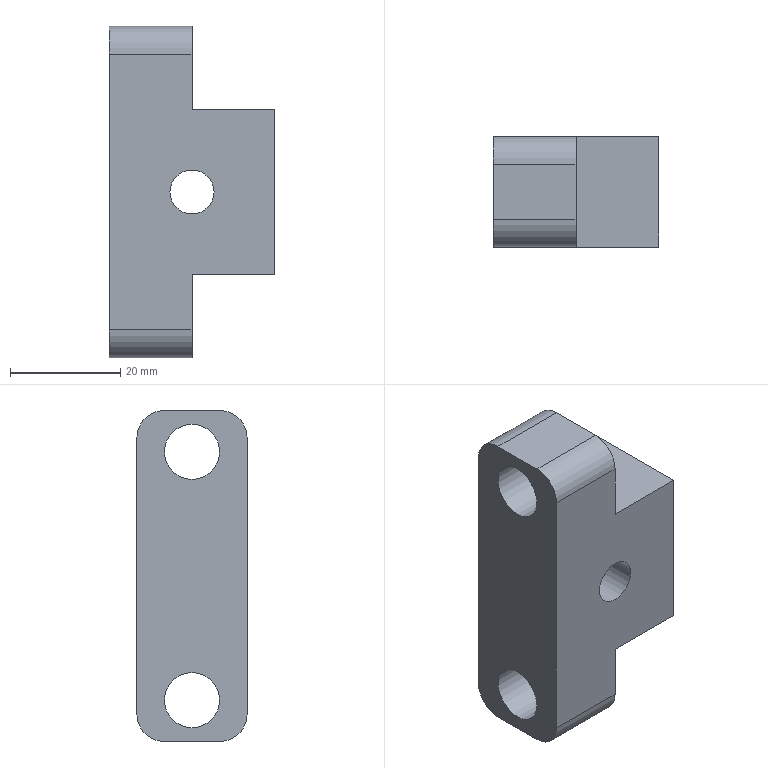Component | NX | FIXED_BASE | 1 solid | 21 faces | volume 22450 mm3 | plane 12 | cylinder 9 | commonest cylinder face diameters 10 x6 13 x2 8 x1